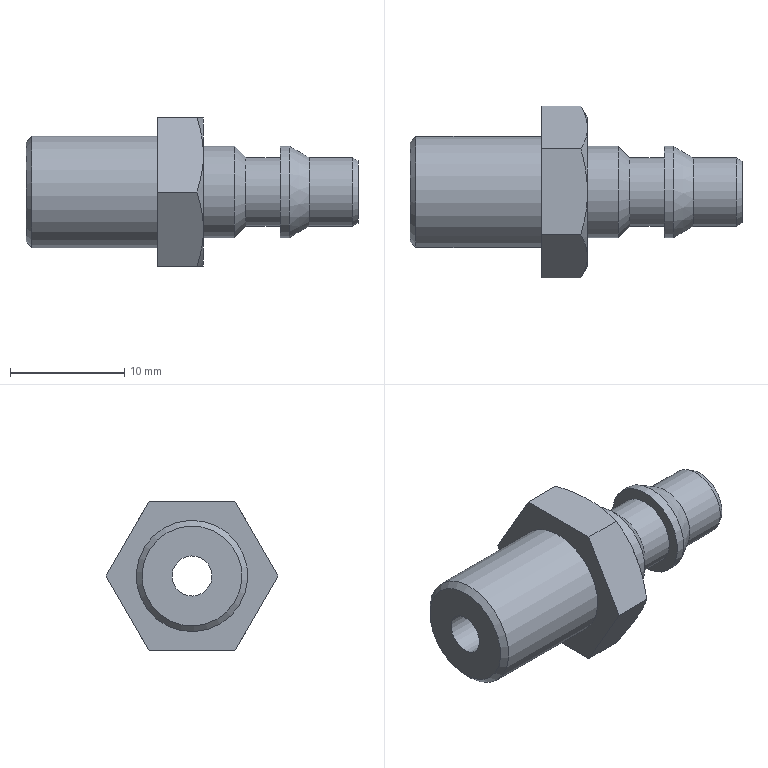Component | NX | TUBE_FITTING | 1 solid | 27 faces | volume 1641 mm3 | plane 11 | cone 10 | cylinder 6 | commonest cylinder face diameters 8 x2 6 x2 9.728 x1 3.5 x1